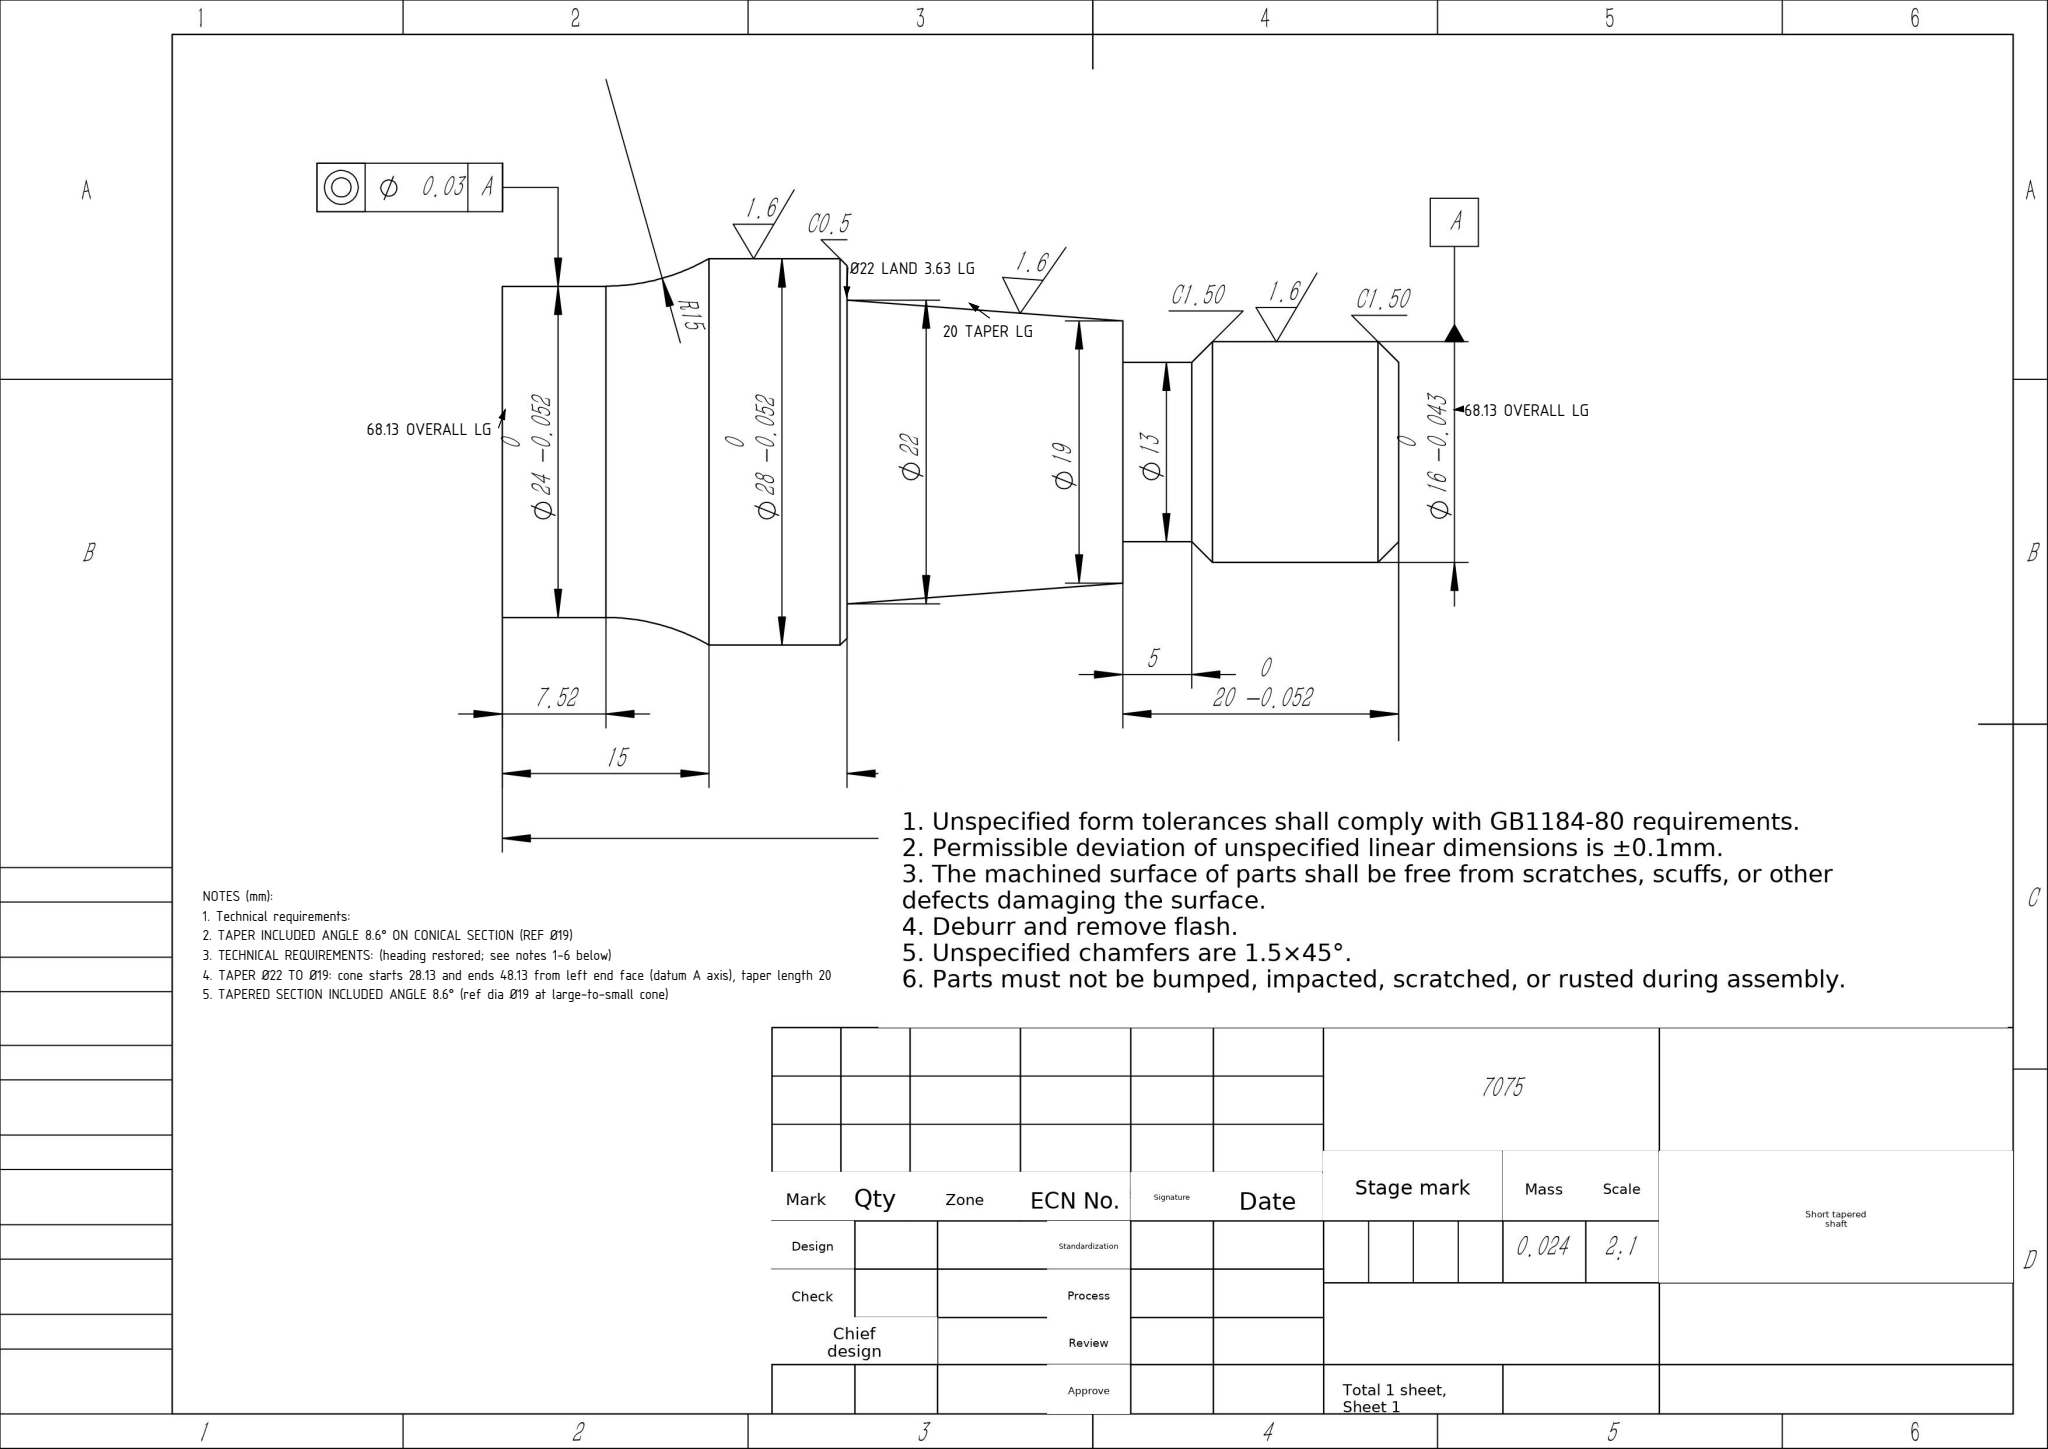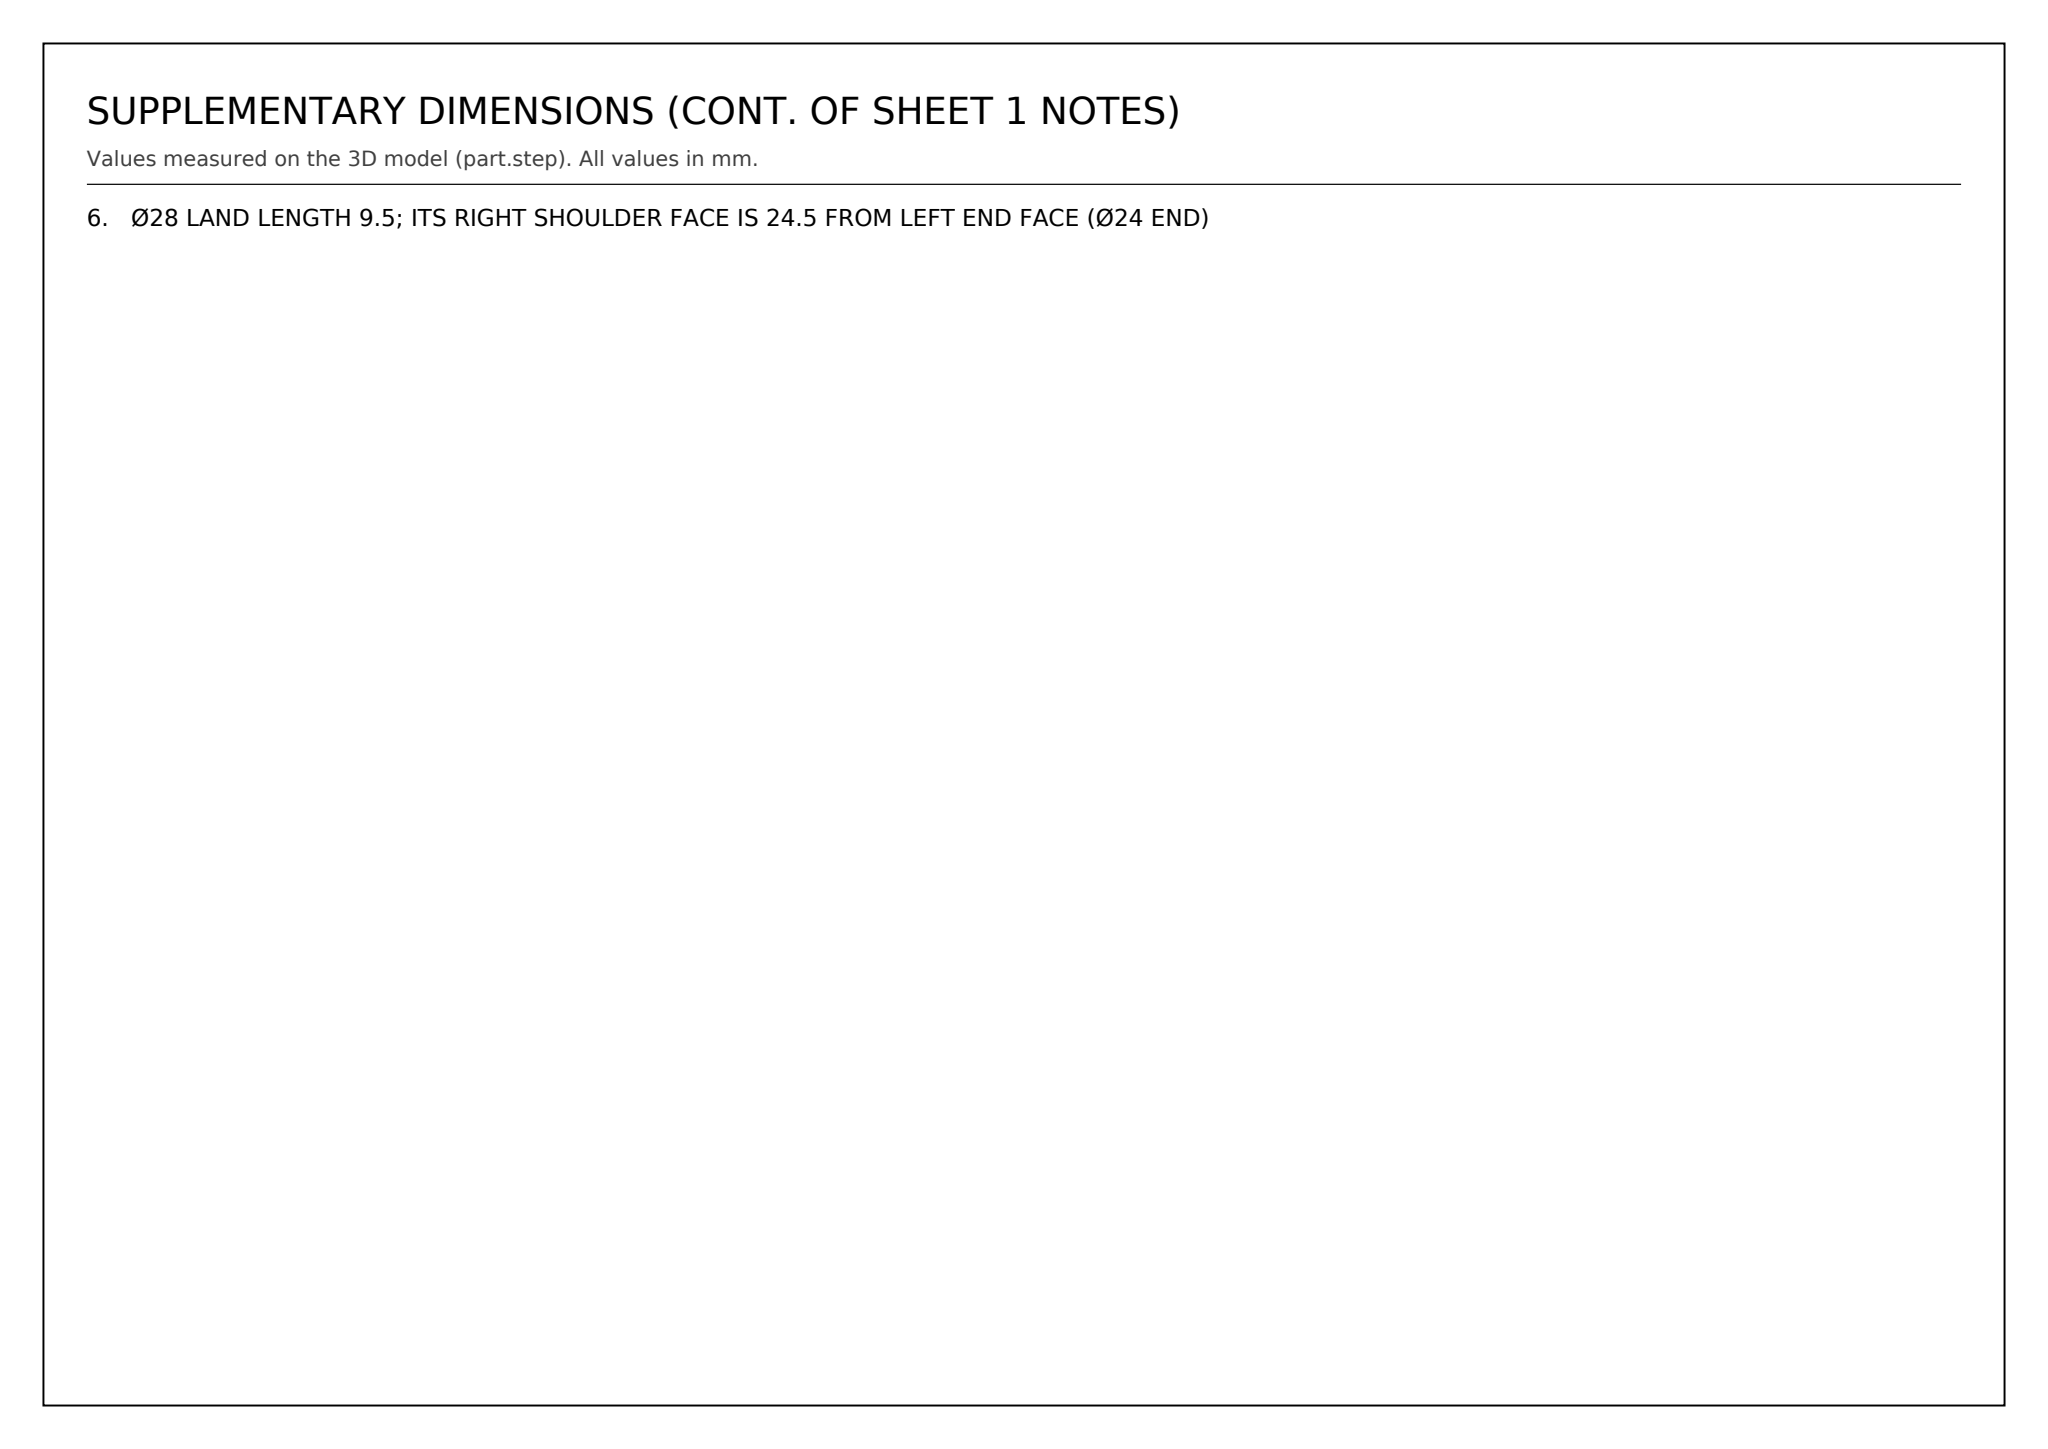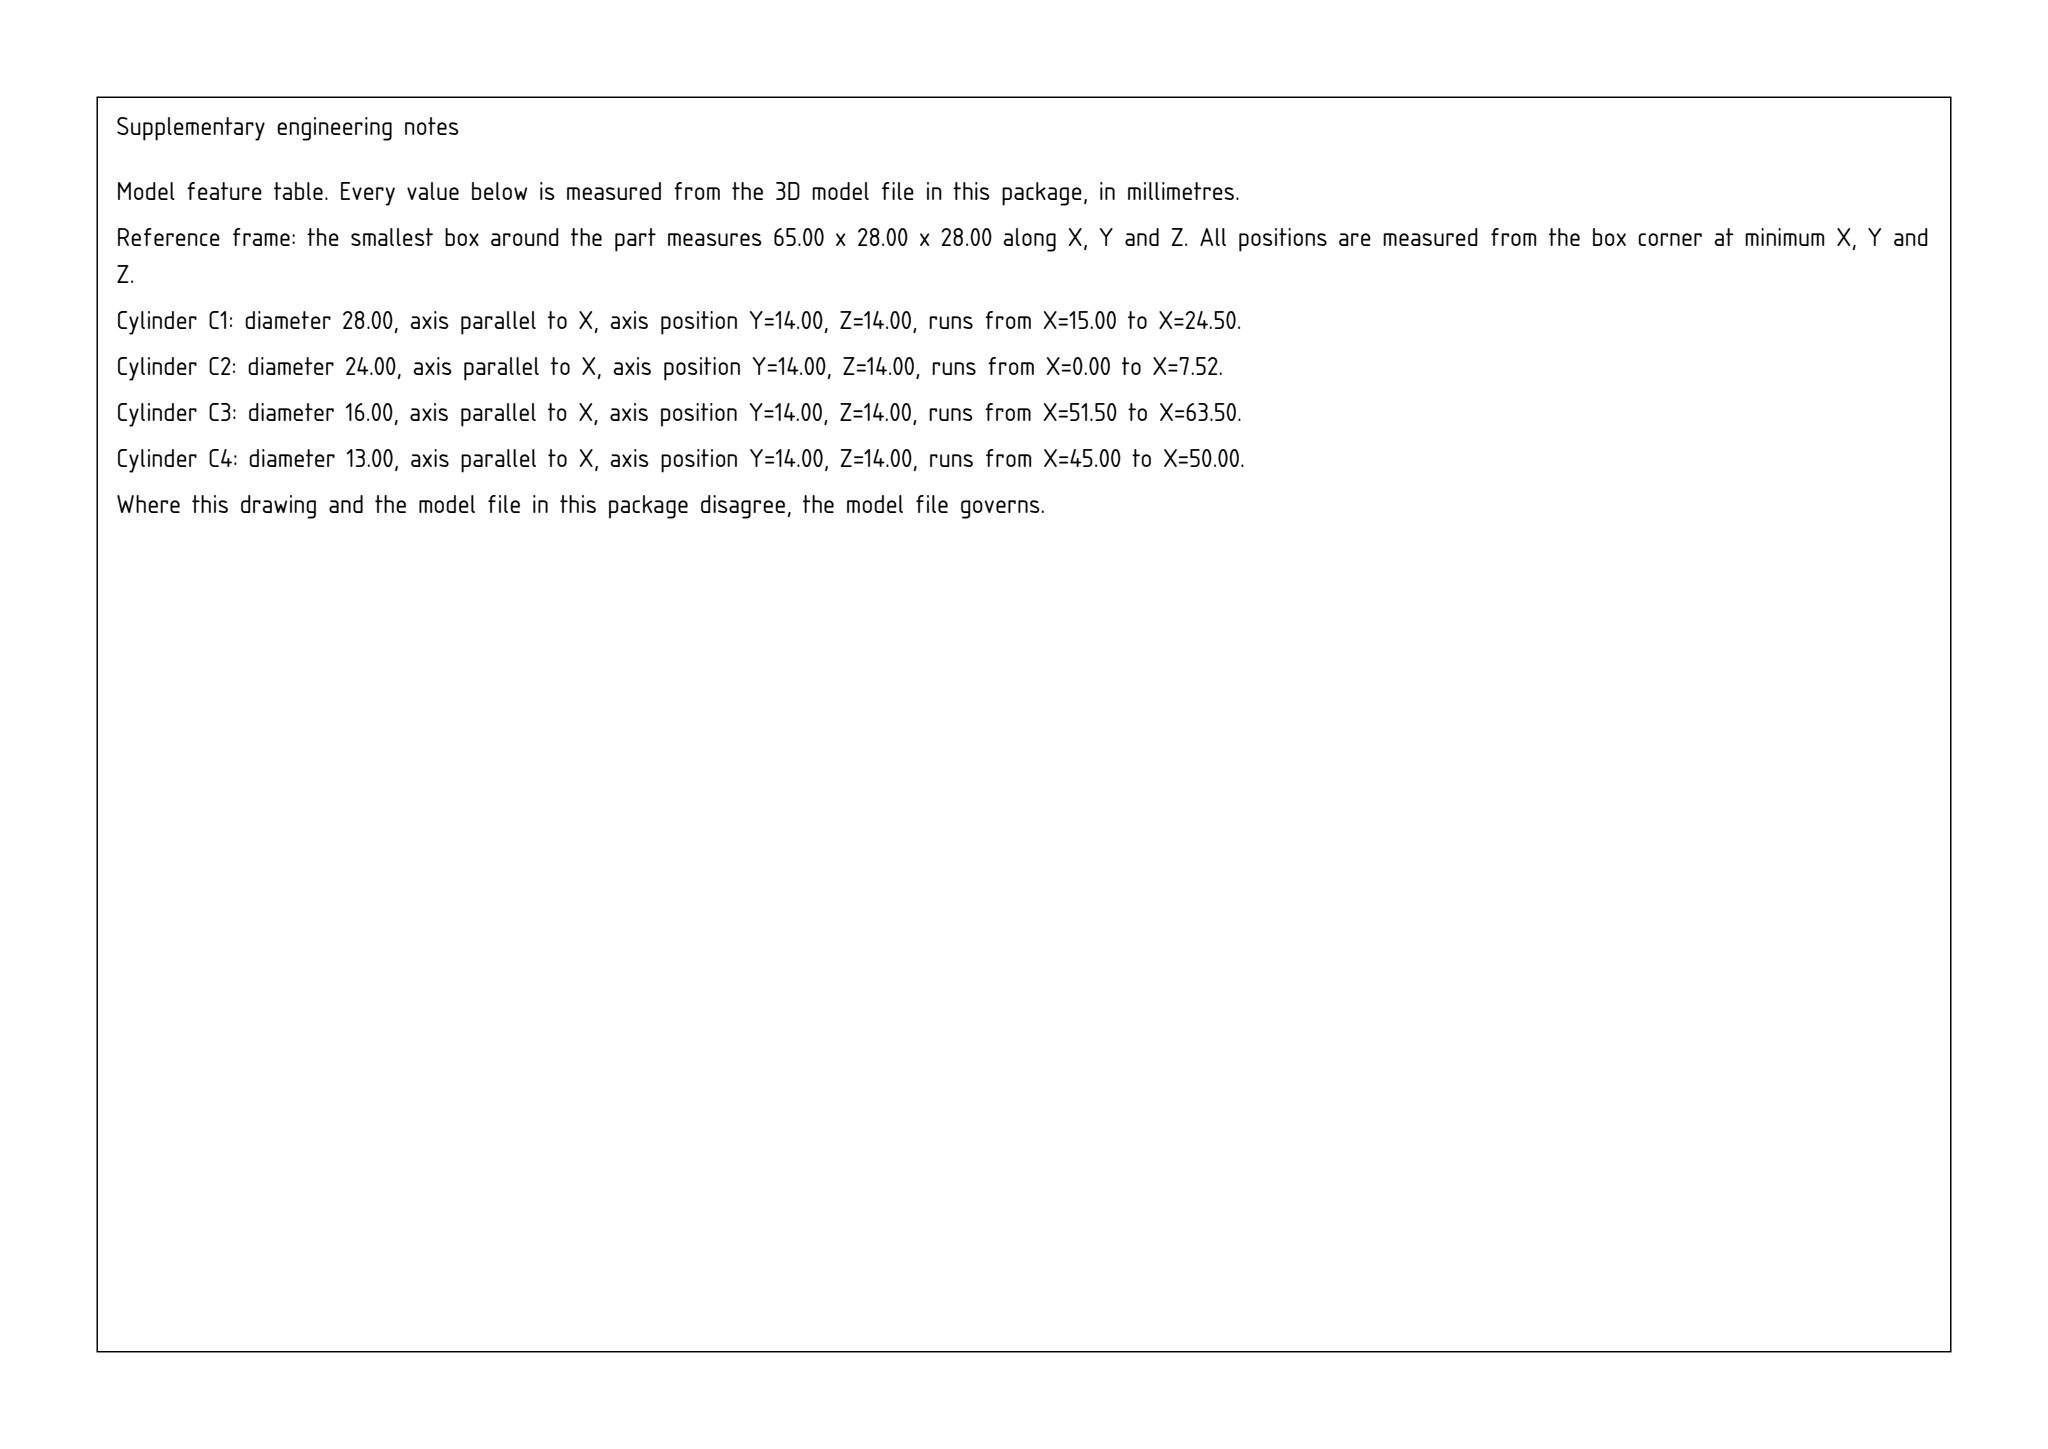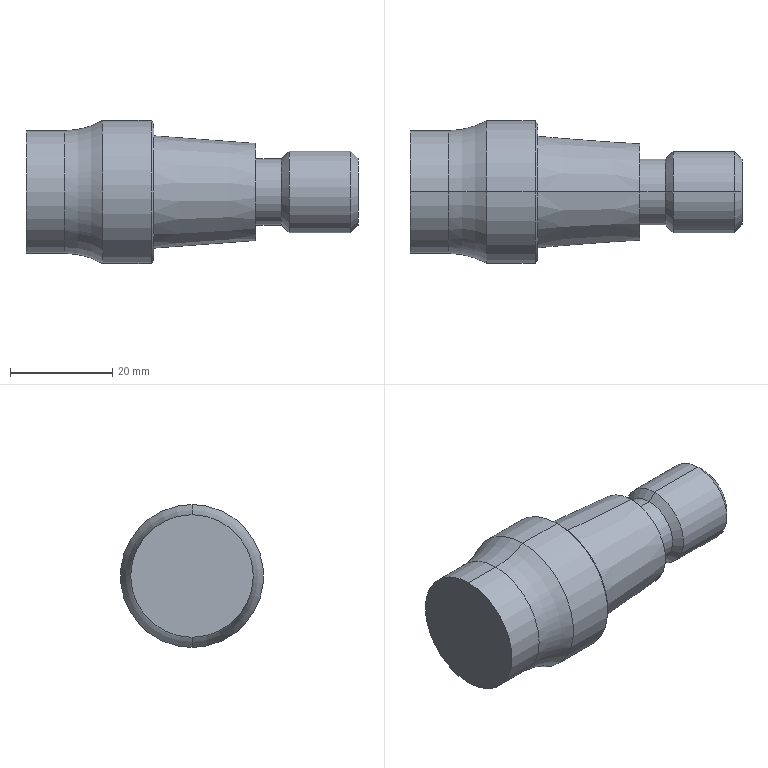Part | SolidWorks | mm | material 7075 | 1 solid | 22 faces | box 65 x 28 x 28 mm | volume 23503 mm3 | cone 8 | cylinder 8 | plane 4 | torus 2 | commonest cylinder face diameters 16 x2 13 x2 28 x2 24 x2
Drawing notes:
Technical requirements: | from the solid: heading text restored after removing merged dimension values (no STEP value)
OVERALL LENGTH 68.13 FROM LEFT END FACE (Ø24 END) TO RIGHT END FACE | from the solid: bbox_xyz x = 68.133; axis_planes x offsets 3.13 ... 68.13
TAPERED SECTION Ø22 TO Ø19: AXIAL LENGTH 20, STARTS 28.13 AND ENDS 48.13 FROM LEFT END FACE | from the solid: axis_planes[x,28.13] and axis_planes[x,48.13]; cone ref_dia 19
TAPER INCLUDED ANGLE 8.6° ON CONICAL SECTION (REF Ø19) | from the solid: cones[included_angle,ref_dia] = [8.6, 19.0]
TECHNICAL REQUIREMENTS: (heading restored; see notes 1-6 below) | from the solid: heading text only - restores garbled line, no dimension value
OVERALL LENGTH 68.13 from left (Ø24) end face to right (Ø16) end face | from the solid: bbox_xyz x = 68.133
TAPER Ø22 TO Ø19: cone starts 28.13 and ends 48.13 from left end face (datum A axis), taper length 20 | from the solid: axis_planes x = 28.13 and x = 48.13 (positions from min corner)
TAPERED SECTION INCLUDED ANGLE 8.6° (ref dia Ø19 at large-to-small cone) | from the solid: cones[included_angle,ref_dia] = [8.6, 19.0]
Ø28 LAND LENGTH 9.5; ITS RIGHT SHOULDER FACE IS 24.5 FROM LEFT END FACE (Ø24 END) | from the solid: cylinders: [28.0,'x',length 9.5] starting 15 from left end face (Ø24 cyl length 7.52 + R15 fillet run), giving shoulder at 24.5
Ø22 LAND FROM 24.5 TO 28.13 FROM LEFT END FACE, LENGTH 3.63, ENDING AT START OF Ø22-TO-Ø19 TAPER | from the solid: axis_planes x=28.13 (cone start) minus Ø28 land end 24.5 (15 + 9.5 Ø28 length)
STEP:
#1=CARTESIAN_POINT('',(25.,0.,-13.5));
#2=VERTEX_POINT('',#1);
#3=CARTESIAN_POINT('',(25.,0.,13.5));
#4=VERTEX_POINT('',#3);
#5=CARTESIAN_POINT('',(25.,0.,0.));
#6=DIRECTION('',(1.,0.,0.));
#7=DIRECTION('',(0.,0.,-1.));
#8=AXIS2_PLACEMENT_3D('',#5,#6,#7);
#9=CIRCLE('',#8,13.5);
#10=EDGE_CURVE('',#2,#4,#9,.T.);
#11=ORIENTED_EDGE('',*,*,#10,.F.);
#12=CARTESIAN_POINT('',(24.5,0.,-14.));
#13=VERTEX_POINT('',#12);
#14=CARTESIAN_POINT('',(25.,0.,-13.5));
#15=DIRECTION('',(-0.7071,0.,-0.7071));
#16=VECTOR('',#15,1000.);
#17=LINE('',#14,#16);
#18=EDGE_CURVE('',#2,#13,#17,.T.);
#19=ORIENTED_EDGE('',*,*,#18,.T.);
#20=CARTESIAN_POINT('',(24.5,0.,14.));
#21=VERTEX_POINT('',#20);
#22=CARTESIAN_POINT('',(24.5,0.,0.));
#23=DIRECTION('',(-1.,0.,0.));
#24=DIRECTION('',(0.,0.,-1.));
#25=AXIS2_PLACEMENT_3D('',#22,#23,#24);
#26=CIRCLE('',#25,14.);
#27=EDGE_CURVE('',#21,#13,#26,.T.);
#28=ORIENTED_EDGE('',*,*,#27,.F.);
#29=CARTESIAN_POINT('',(25.,0.,13.5));
#30=DIRECTION('',(-0.7071,0.,0.7071));
#31=VECTOR('',#30,1000.);
#32=LINE('',#29,#31);
#33=EDGE_CURVE('',#4,#21,#32,.T.);
#34=ORIENTED_EDGE('',*,*,#33,.F.);
#35=EDGE_LOOP('',(#11,#19,#28,#34));
#36=FACE_OUTER_BOUND('',#35,.T.);
#37=CARTESIAN_POINT('',(25.,0.,0.));
#38=DIRECTION('',(-1.,0.,0.));
#39=DIRECTION('',(0.,0.,1.));
#40=AXIS2_PLACEMENT_3D('',#37,#38,#39);
#41=CONICAL_SURFACE('',#40,13.5,0.7854);
#42=ADVANCED_FACE('',(#36),#41,.T.);
#43=CARTESIAN_POINT('',(65.,0.,-6.5));
#44=VERTEX_POINT('',#43);
#45=CARTESIAN_POINT('',(65.,0.,6.5));
#46=VERTEX_POINT('',#45);
#47=CARTESIAN_POINT('',(65.,0.,0.));
#48=DIRECTION('',(1.,0.,0.));
#49=DIRECTION('',(0.,0.,-1.));
#50=AXIS2_PLACEMENT_3D('',#47,#48,#49);
#51=CIRCLE('',#50,6.5);
#52=EDGE_CURVE('',#44,#46,#51,.T.);
#53=ORIENTED_EDGE('',*,*,#52,.F.);
#54=CARTESIAN_POINT('',(63.5,0.,-8.));
#55=VERTEX_POINT('',#54);
#56=CARTESIAN_POINT('',(65.,0.,-6.5));
#57=DIRECTION('',(-0.7071,0.,-0.7071));
#58=VECTOR('',#57,1000.);
#59=LINE('',#56,#58);
#60=EDGE_CURVE('',#44,#55,#59,.T.);
#61=ORIENTED_EDGE('',*,*,#60,.T.);
#62=CARTESIAN_POINT('',(63.5,0.,8.));
#63=VERTEX_POINT('',#62);
#64=CARTESIAN_POINT('',(63.5,0.,0.));
#65=DIRECTION('',(-1.,0.,0.));
#66=DIRECTION('',(0.,0.,-1.));
#67=AXIS2_PLACEMENT_3D('',#64,#65,#66);
#68=CIRCLE('',#67,8.);
#69=EDGE_CURVE('',#63,#55,#68,.T.);
#70=ORIENTED_EDGE('',*,*,#69,.F.);
#71=CARTESIAN_POINT('',(65.,0.,6.5));
#72=DIRECTION('',(-0.7071,0.,0.7071));
#73=VECTOR('',#72,1000.);
#74=LINE('',#71,#73);
#75=EDGE_CURVE('',#46,#63,#74,.T.);
#76=ORIENTED_EDGE('',*,*,#75,.F.);
#77=EDGE_LOOP('',(#53,#61,#70,#76));
#78=FACE_OUTER_BOUND('',#77,.T.);
#79=CARTESIAN_POINT('',(65.,0.,0.));
#80=DIRECTION('',(-1.,0.,0.));
#81=DIRECTION('',(0.,0.,1.));
#82=AXIS2_PLACEMENT_3D('',#79,#80,#81);
#83=CONICAL_SURFACE('',#82,6.5,0.7854);
#84=ADVANCED_FACE('',(#78),#83,.T.);
#85=CARTESIAN_POINT('',(50.,0.,-6.5));
#86=VERTEX_POINT('',#85);
#87=CARTESIAN_POINT('',(50.,0.,6.5));
#88=VERTEX_POINT('',#87);
#89=CARTESIAN_POINT('',(50.,0.,0.));
#90=DIRECTION('',(1.,0.,0.));
#91=DIRECTION('',(0.,0.,-1.));
#92=AXIS2_PLACEMENT_3D('',#89,#90,#91);
#93=CIRCLE('',#92,6.5);
#94=EDGE_CURVE('',#86,#88,#93,.T.);
#95=ORIENTED_EDGE('',*,*,#94,.T.);
#96=CARTESIAN_POINT('',(51.5,0.,8.));
#97=VERTEX_POINT('',#96);
#98=CARTESIAN_POINT('',(51.5,0.,8.));
#99=DIRECTION('',(0.7071,0.,0.7071));
#100=VECTOR('',#99,1000.);
#101=LINE('',#98,#100);
#102=EDGE_CURVE('',#88,#97,#101,.T.);
#103=ORIENTED_EDGE('',*,*,#102,.T.);
#104=CARTESIAN_POINT('',(51.5,0.,-8.));
#105=VERTEX_POINT('',#104);
#106=CARTESIAN_POINT('',(51.5,0.,0.));
#107=DIRECTION('',(1.,0.,0.));
#108=DIRECTION('',(0.,0.,1.));
#109=AXIS2_PLACEMENT_3D('',#106,#107,#108);
#110=CIRCLE('',#109,8.);
#111=EDGE_CURVE('',#105,#97,#110,.T.);
#112=ORIENTED_EDGE('',*,*,#111,.F.);
#113=CARTESIAN_POINT('',(51.5,0.,-8.));
#114=DIRECTION('',(0.7071,0.,-0.7071));
#115=VECTOR('',#114,1000.);
#116=LINE('',#113,#115);
#117=EDGE_CURVE('',#86,#105,#116,.T.);
#118=ORIENTED_EDGE('',*,*,#117,.F.);
#119=EDGE_LOOP('',(#95,#103,#112,#118));
#120=FACE_OUTER_BOUND('',#119,.T.);
#121=CARTESIAN_POINT('',(51.5,0.,0.));
#122=DIRECTION('',(1.,0.,0.));
#123=DIRECTION('',(0.,0.,-1.));
#124=AXIS2_PLACEMENT_3D('',#121,#122,#123);
#125=CONICAL_SURFACE('',#124,8.,0.7854);
#126=ADVANCED_FACE('',(#120),#125,.T.);
#127=ORIENTED_EDGE('',*,*,#111,.T.);
#128=CARTESIAN_POINT('',(65.,0.,8.));
#129=DIRECTION('',(1.,0.,0.));
#130=VECTOR('',#129,1000.);
#131=LINE('',#128,#130);
#132=EDGE_CURVE('',#97,#63,#131,.T.);
#133=ORIENTED_EDGE('',*,*,#132,.T.);
#134=ORIENTED_EDGE('',*,*,#69,.T.);
#135=CARTESIAN_POINT('',(65.,0.,-8.));
#136=DIRECTION('',(1.,0.,0.));
#137=VECTOR('',#136,1000.);
#138=LINE('',#135,#137);
#139=EDGE_CURVE('',#105,#55,#138,.T.);
#140=ORIENTED_EDGE('',*,*,#139,.F.);
#141=EDGE_LOOP('',(#127,#133,#134,#140));
#142=FACE_OUTER_BOUND('',#141,.T.);
#143=CARTESIAN_POINT('',(65.,0.,0.));
#144=DIRECTION('',(1.,0.,0.));
#145=DIRECTION('',(0.,0.,-1.));
#146=AXIS2_PLACEMENT_3D('',#143,#144,#145);
#147=CYLINDRICAL_SURFACE('',#146,8.);
#148=ADVANCED_FACE('',(#142),#147,.T.);
#149=CARTESIAN_POINT('',(45.,0.,-6.5));
#150=VERTEX_POINT('',#149);
#151=CARTESIAN_POINT('',(45.,0.,6.5));
#152=VERTEX_POINT('',#151);
#153=CARTESIAN_POINT('',(45.,0.,0.));
#154=DIRECTION('',(1.,0.,0.));
#155=DIRECTION('',(0.,0.,-1.));
#156=AXIS2_PLACEMENT_3D('',#153,#154,#155);
#157=CIRCLE('',#156,6.5);
#158=EDGE_CURVE('',#150,#152,#157,.T.);
#159=ORIENTED_EDGE('',*,*,#158,.T.);
#160=CARTESIAN_POINT('',(65.,0.,6.5));
#161=DIRECTION('',(1.,0.,0.));
#162=VECTOR('',#161,1000.);
#163=LINE('',#160,#162);
#164=EDGE_CURVE('',#152,#88,#163,.T.);
#165=ORIENTED_EDGE('',*,*,#164,.T.);
#166=ORIENTED_EDGE('',*,*,#94,.F.);
#167=CARTESIAN_POINT('',(65.,0.,-6.5));
#168=DIRECTION('',(1.,0.,0.));
#169=VECTOR('',#168,1000.);
#170=LINE('',#167,#169);
#171=EDGE_CURVE('',#150,#86,#170,.T.);
#172=ORIENTED_EDGE('',*,*,#171,.F.);
#173=EDGE_LOOP('',(#159,#165,#166,#172));
#174=FACE_OUTER_BOUND('',#173,.T.);
#175=CARTESIAN_POINT('',(65.,0.,0.));
#176=DIRECTION('',(1.,0.,0.));
#177=DIRECTION('',(0.,0.,-1.));
#178=AXIS2_PLACEMENT_3D('',#175,#176,#177);
#179=CYLINDRICAL_SURFACE('',#178,6.5);
#180=ADVANCED_FACE('',(#174),#179,.T.);
#181=CARTESIAN_POINT('',(45.,0.,-9.5));
#182=VERTEX_POINT('',#181);
#183=CARTESIAN_POINT('',(45.,0.,9.5));
#184=VERTEX_POINT('',#183);
#185=CARTESIAN_POINT('',(45.,0.,0.));
#186=DIRECTION('',(1.,0.,0.));
#187=DIRECTION('',(0.,0.,-1.));
#188=AXIS2_PLACEMENT_3D('',#185,#186,#187);
#189=CIRCLE('',#188,9.5);
#190=EDGE_CURVE('',#182,#184,#189,.T.);
#191=ORIENTED_EDGE('',*,*,#190,.F.);
#192=CARTESIAN_POINT('',(25.,0.,-11.));
#193=VERTEX_POINT('',#192);
#194=CARTESIAN_POINT('',(45.,0.,-9.5));
#195=DIRECTION('',(-0.9972,0.,-0.07479));
#196=VECTOR('',#195,1000.);
#197=LINE('',#194,#196);
#198=EDGE_CURVE('',#182,#193,#197,.T.);
#199=ORIENTED_EDGE('',*,*,#198,.T.);
#200=CARTESIAN_POINT('',(25.,0.,11.));
#201=VERTEX_POINT('',#200);
#202=CARTESIAN_POINT('',(25.,0.,0.));
#203=DIRECTION('',(1.,0.,0.));
#204=DIRECTION('',(0.,0.,-1.));
#205=AXIS2_PLACEMENT_3D('',#202,#203,#204);
#206=CIRCLE('',#205,11.);
#207=EDGE_CURVE('',#193,#201,#206,.T.);
#208=ORIENTED_EDGE('',*,*,#207,.T.);
#209=CARTESIAN_POINT('',(45.,0.,9.5));
#210=DIRECTION('',(-0.9972,0.,0.07479));
#211=VECTOR('',#210,1000.);
#212=LINE('',#209,#211);
#213=EDGE_CURVE('',#184,#201,#212,.T.);
#214=ORIENTED_EDGE('',*,*,#213,.F.);
#215=EDGE_LOOP('',(#191,#199,#208,#214));
#216=FACE_OUTER_BOUND('',#215,.T.);
#217=CARTESIAN_POINT('',(45.,0.,0.));
#218=DIRECTION('',(-1.,0.,0.));
#219=DIRECTION('',(0.,0.,1.));
#220=AXIS2_PLACEMENT_3D('',#217,#218,#219);
#221=CONICAL_SURFACE('',#220,9.5,0.07486);
#222=ADVANCED_FACE('',(#216),#221,.T.);
#223=CARTESIAN_POINT('',(15.,0.,-14.));
#224=VERTEX_POINT('',#223);
#225=CARTESIAN_POINT('',(15.,0.,14.));
#226=VERTEX_POINT('',#225);
#227=CARTESIAN_POINT('',(15.,0.,0.));
#228=DIRECTION('',(1.,0.,0.));
#229=DIRECTION('',(0.,0.,-1.));
#230=AXIS2_PLACEMENT_3D('',#227,#228,#229);
#231=CIRCLE('',#230,14.);
#232=EDGE_CURVE('',#224,#226,#231,.T.);
#233=ORIENTED_EDGE('',*,*,#232,.T.);
#234=CARTESIAN_POINT('',(65.,0.,14.));
#235=DIRECTION('',(1.,0.,0.));
#236=VECTOR('',#235,1000.);
#237=LINE('',#234,#236);
#238=EDGE_CURVE('',#226,#21,#237,.T.);
#239=ORIENTED_EDGE('',*,*,#238,.T.);
#240=ORIENTED_EDGE('',*,*,#27,.T.);
#241=CARTESIAN_POINT('',(65.,0.,-14.));
#242=DIRECTION('',(1.,0.,0.));
#243=VECTOR('',#242,1000.);
#244=LINE('',#241,#243);
#245=EDGE_CURVE('',#224,#13,#244,.T.);
#246=ORIENTED_EDGE('',*,*,#245,.F.);
#247=EDGE_LOOP('',(#233,#239,#240,#246));
#248=FACE_OUTER_BOUND('',#247,.T.);
#249=CARTESIAN_POINT('',(65.,0.,0.));
#250=DIRECTION('',(1.,0.,0.));
#251=DIRECTION('',(0.,0.,-1.));
#252=AXIS2_PLACEMENT_3D('',#249,#250,#251);
#253=CYLINDRICAL_SURFACE('',#252,14.);
#254=ADVANCED_FACE('',(#248),#253,.T.);
#255=CARTESIAN_POINT('',(15.,0.,0.));
#256=DIRECTION('',(1.,0.,0.));
#257=DIRECTION('',(0.,0.,-1.));
#258=AXIS2_PLACEMENT_3D('',#255,#256,#257);
#259=CIRCLE('',#258,14.);
#260=EDGE_CURVE('',#226,#224,#259,.T.);
#261=ORIENTED_EDGE('',*,*,#260,.F.);
#262=CARTESIAN_POINT('',(7.517,0.,12.));
#263=VERTEX_POINT('',#262);
#264=CARTESIAN_POINT('',(7.517,0.,27.));
#265=DIRECTION('',(0.,1.,-0.));
#266=DIRECTION('',(0.,0.,1.));
#267=AXIS2_PLACEMENT_3D('',#264,#265,#266);
#268=CIRCLE('',#267,15.);
#269=EDGE_CURVE('',#226,#263,#268,.T.);
#270=ORIENTED_EDGE('',*,*,#269,.T.);
#271=CARTESIAN_POINT('',(7.517,0.,-12.));
#272=VERTEX_POINT('',#271);
#273=CARTESIAN_POINT('',(7.517,0.,0.));
#274=DIRECTION('',(1.,0.,0.));
#275=DIRECTION('',(0.,0.,-1.));
#276=AXIS2_PLACEMENT_3D('',#273,#274,#275);
#277=CIRCLE('',#276,12.);
#278=EDGE_CURVE('',#263,#272,#277,.T.);
#279=ORIENTED_EDGE('',*,*,#278,.T.);
#280=CARTESIAN_POINT('',(7.517,0.,-27.));
#281=DIRECTION('',(0.,-1.,0.));
#282=DIRECTION('',(0.,0.,-1.));
#283=AXIS2_PLACEMENT_3D('',#280,#281,#282);
#284=CIRCLE('',#283,15.);
#285=EDGE_CURVE('',#224,#272,#284,.T.);
#286=ORIENTED_EDGE('',*,*,#285,.F.);
#287=EDGE_LOOP('',(#261,#270,#279,#286));
#288=FACE_OUTER_BOUND('',#287,.T.);
#289=CARTESIAN_POINT('',(7.517,0.,0.));
#290=DIRECTION('',(1.,0.,0.));
#291=DIRECTION('',(0.,0.,-1.));
#292=AXIS2_PLACEMENT_3D('',#289,#290,#291);
#293=TOROIDAL_SURFACE('',#292,27.,15.);
#294=ADVANCED_FACE('',(#288),#293,.F.);
#295=CARTESIAN_POINT('',(0.,0.,-12.));
#296=VERTEX_POINT('',#295);
#297=CARTESIAN_POINT('',(0.,0.,12.));
#298=VERTEX_POINT('',#297);
#299=CARTESIAN_POINT('',(0.,0.,0.));
#300=DIRECTION('',(1.,0.,0.));
#301=DIRECTION('',(0.,0.,-1.));
#302=AXIS2_PLACEMENT_3D('',#299,#300,#301);
#303=CIRCLE('',#302,12.);
#304=EDGE_CURVE('',#296,#298,#303,.T.);
#305=ORIENTED_EDGE('',*,*,#304,.T.);
#306=CARTESIAN_POINT('',(65.,0.,12.));
#307=DIRECTION('',(1.,0.,0.));
#308=VECTOR('',#307,1000.);
#309=LINE('',#306,#308);
#310=EDGE_CURVE('',#298,#263,#309,.T.);
#311=ORIENTED_EDGE('',*,*,#310,.T.);
#312=CARTESIAN_POINT('',(7.517,0.,0.));
#313=DIRECTION('',(1.,0.,0.));
#314=DIRECTION('',(0.,0.,-1.));
#315=AXIS2_PLACEMENT_3D('',#312,#313,#314);
#316=CIRCLE('',#315,12.);
#317=EDGE_CURVE('',#272,#263,#316,.T.);
#318=ORIENTED_EDGE('',*,*,#317,.F.);
#319=CARTESIAN_POINT('',(65.,0.,-12.));
#320=DIRECTION('',(1.,0.,0.));
#321=VECTOR('',#320,1000.);
#322=LINE('',#319,#321);
#323=EDGE_CURVE('',#296,#272,#322,.T.);
#324=ORIENTED_EDGE('',*,*,#323,.F.);
#325=EDGE_LOOP('',(#305,#311,#318,#324));
#326=FACE_OUTER_BOUND('',#325,.T.);
#327=CARTESIAN_POINT('',(65.,0.,0.));
#328=DIRECTION('',(1.,0.,0.));
#329=DIRECTION('',(0.,0.,-1.));
#330=AXIS2_PLACEMENT_3D('',#327,#328,#329);
#331=CYLINDRICAL_SURFACE('',#330,12.);
#332=ADVANCED_FACE('',(#326),#331,.T.);
#333=ORIENTED_EDGE('',*,*,#304,.F.);
#334=CARTESIAN_POINT('',(0.,0.,0.));
#335=DIRECTION('',(1.,0.,0.));
#336=DIRECTION('',(0.,0.,-1.));
#337=AXIS2_PLACEMENT_3D('',#334,#335,#336);
#338=CIRCLE('',#337,12.);
#339=EDGE_CURVE('',#298,#296,#338,.T.);
#340=ORIENTED_EDGE('',*,*,#339,.F.);
#341=EDGE_LOOP('',(#333,#340));
#342=FACE_OUTER_BOUND('',#341,.T.);
#343=CARTESIAN_POINT('',(0.,0.,0.));
#344=DIRECTION('',(-1.,0.,0.));
#345=DIRECTION('',(0.,0.,1.));
#346=AXIS2_PLACEMENT_3D('',#343,#344,#345);
#347=PLANE('',#346);
#348=ADVANCED_FACE('',(#342),#347,.T.);
#349=ORIENTED_EDGE('',*,*,#310,.F.);
#350=ORIENTED_EDGE('',*,*,#339,.T.);
#351=ORIENTED_EDGE('',*,*,#323,.T.);
#352=ORIENTED_EDGE('',*,*,#278,.F.);
#353=EDGE_LOOP('',(#349,#350,#351,#352));
#354=FACE_OUTER_BOUND('',#353,.T.);
#355=CARTESIAN_POINT('',(65.,0.,0.));
#356=DIRECTION('',(1.,0.,0.));
#357=DIRECTION('',(0.,0.,-1.));
#358=AXIS2_PLACEMENT_3D('',#355,#356,#357);
#359=CYLINDRICAL_SURFACE('',#358,12.);
#360=ADVANCED_FACE('',(#354),#359,.T.);
#361=ORIENTED_EDGE('',*,*,#269,.F.);
#362=ORIENTED_EDGE('',*,*,#232,.F.);
#363=ORIENTED_EDGE('',*,*,#285,.T.);
#364=ORIENTED_EDGE('',*,*,#317,.T.);
#365=EDGE_LOOP('',(#361,#362,#363,#364));
#366=FACE_OUTER_BOUND('',#365,.T.);
#367=CARTESIAN_POINT('',(7.517,0.,0.));
#368=DIRECTION('',(1.,0.,0.));
#369=DIRECTION('',(0.,0.,-1.));
#370=AXIS2_PLACEMENT_3D('',#367,#368,#369);
#371=TOROIDAL_SURFACE('',#370,27.,15.);
#372=ADVANCED_FACE('',(#366),#371,.F.);
#373=ORIENTED_EDGE('',*,*,#238,.F.);
#374=ORIENTED_EDGE('',*,*,#260,.T.);
#375=ORIENTED_EDGE('',*,*,#245,.T.);
#376=CARTESIAN_POINT('',(24.5,0.,0.));
#377=DIRECTION('',(-1.,0.,0.));
#378=DIRECTION('',(0.,0.,-1.));
#379=AXIS2_PLACEMENT_3D('',#376,#377,#378);
#380=CIRCLE('',#379,14.);
#381=EDGE_CURVE('',#13,#21,#380,.T.);
#382=ORIENTED_EDGE('',*,*,#381,.T.);
#383=EDGE_LOOP('',(#373,#374,#375,#382));
#384=FACE_OUTER_BOUND('',#383,.T.);
#385=CARTESIAN_POINT('',(65.,0.,0.));
#386=DIRECTION('',(1.,0.,0.));
#387=DIRECTION('',(0.,0.,-1.));
#388=AXIS2_PLACEMENT_3D('',#385,#386,#387);
#389=CYLINDRICAL_SURFACE('',#388,14.);
#390=ADVANCED_FACE('',(#384),#389,.T.);
#391=CARTESIAN_POINT('',(25.,0.,0.));
#392=DIRECTION('',(1.,0.,0.));
#393=DIRECTION('',(0.,0.,-1.));
#394=AXIS2_PLACEMENT_3D('',#391,#392,#393);
#395=CIRCLE('',#394,13.5);
#396=EDGE_CURVE('',#4,#2,#395,.T.);
#397=ORIENTED_EDGE('',*,*,#396,.T.);
#398=ORIENTED_EDGE('',*,*,#10,.T.);
#399=EDGE_LOOP('',(#397,#398));
#400=FACE_OUTER_BOUND('',#399,.T.);
#401=CARTESIAN_POINT('',(25.,0.,0.));
#402=DIRECTION('',(1.,0.,0.));
#403=DIRECTION('',(0.,0.,-1.));
#404=AXIS2_PLACEMENT_3D('',#401,#402,#403);
#405=CIRCLE('',#404,11.);
#406=EDGE_CURVE('',#201,#193,#405,.T.);
#407=ORIENTED_EDGE('',*,*,#406,.F.);
#408=ORIENTED_EDGE('',*,*,#207,.F.);
#409=EDGE_LOOP('',(#407,#408));
#410=FACE_BOUND('',#409,.T.);
#411=CARTESIAN_POINT('',(25.,14.,0.));
#412=DIRECTION('',(1.,0.,0.));
#413=DIRECTION('',(0.,0.,-1.));
#414=AXIS2_PLACEMENT_3D('',#411,#412,#413);
#415=PLANE('',#414);
#416=ADVANCED_FACE('',(#400,#410),#415,.T.);
#417=ORIENTED_EDGE('',*,*,#198,.F.);
#418=CARTESIAN_POINT('',(45.,0.,0.));
#419=DIRECTION('',(1.,0.,0.));
#420=DIRECTION('',(0.,0.,-1.));
#421=AXIS2_PLACEMENT_3D('',#418,#419,#420);
#422=CIRCLE('',#421,9.5);
#423=EDGE_CURVE('',#184,#182,#422,.T.);
#424=ORIENTED_EDGE('',*,*,#423,.F.);
#425=ORIENTED_EDGE('',*,*,#213,.T.);
#426=ORIENTED_EDGE('',*,*,#406,.T.);
#427=EDGE_LOOP('',(#417,#424,#425,#426));
#428=FACE_OUTER_BOUND('',#427,.T.);
#429=CARTESIAN_POINT('',(45.,0.,0.));
#430=DIRECTION('',(-1.,0.,0.));
#431=DIRECTION('',(0.,0.,1.));
#432=AXIS2_PLACEMENT_3D('',#429,#430,#431);
#433=CONICAL_SURFACE('',#432,9.5,0.07486);
#434=ADVANCED_FACE('',(#428),#433,.T.);
#435=ORIENTED_EDGE('',*,*,#423,.T.);
#436=ORIENTED_EDGE('',*,*,#190,.T.);
#437=EDGE_LOOP('',(#435,#436));
#438=FACE_OUTER_BOUND('',#437,.T.);
#439=ORIENTED_EDGE('',*,*,#158,.F.);
#440=CARTESIAN_POINT('',(45.,0.,0.));
#441=DIRECTION('',(1.,0.,0.));
#442=DIRECTION('',(0.,0.,-1.));
#443=AXIS2_PLACEMENT_3D('',#440,#441,#442);
#444=CIRCLE('',#443,6.5);
#445=EDGE_CURVE('',#152,#150,#444,.T.);
#446=ORIENTED_EDGE('',*,*,#445,.F.);
#447=EDGE_LOOP('',(#439,#446));
#448=FACE_BOUND('',#447,.T.);
#449=CARTESIAN_POINT('',(45.,9.5,0.));
#450=DIRECTION('',(1.,0.,0.));
#451=DIRECTION('',(0.,0.,-1.));
#452=AXIS2_PLACEMENT_3D('',#449,#450,#451);
#453=PLANE('',#452);
#454=ADVANCED_FACE('',(#438,#448),#453,.T.);
#455=ORIENTED_EDGE('',*,*,#164,.F.);
#456=ORIENTED_EDGE('',*,*,#445,.T.);
#457=ORIENTED_EDGE('',*,*,#171,.T.);
#458=CARTESIAN_POINT('',(50.,0.,0.));
#459=DIRECTION('',(1.,0.,0.));
#460=DIRECTION('',(0.,0.,-1.));
#461=AXIS2_PLACEMENT_3D('',#458,#459,#460);
#462=CIRCLE('',#461,6.5);
#463=EDGE_CURVE('',#88,#86,#462,.T.);
#464=ORIENTED_EDGE('',*,*,#463,.F.);
#465=EDGE_LOOP('',(#455,#456,#457,#464));
#466=FACE_OUTER_BOUND('',#465,.T.);
#467=CARTESIAN_POINT('',(65.,0.,0.));
#468=DIRECTION('',(1.,0.,0.));
#469=DIRECTION('',(0.,0.,-1.));
#470=AXIS2_PLACEMENT_3D('',#467,#468,#469);
#471=CYLINDRICAL_SURFACE('',#470,6.5);
#472=ADVANCED_FACE('',(#466),#471,.T.);
#473=ORIENTED_EDGE('',*,*,#132,.F.);
#474=CARTESIAN_POINT('',(51.5,0.,0.));
#475=DIRECTION('',(1.,0.,0.));
#476=DIRECTION('',(0.,0.,1.));
#477=AXIS2_PLACEMENT_3D('',#474,#475,#476);
#478=CIRCLE('',#477,8.);
#479=EDGE_CURVE('',#97,#105,#478,.T.);
#480=ORIENTED_EDGE('',*,*,#479,.T.);
#481=ORIENTED_EDGE('',*,*,#139,.T.);
#482=CARTESIAN_POINT('',(63.5,0.,0.));
#483=DIRECTION('',(-1.,0.,0.));
#484=DIRECTION('',(0.,0.,-1.));
#485=AXIS2_PLACEMENT_3D('',#482,#483,#484);
#486=CIRCLE('',#485,8.);
#487=EDGE_CURVE('',#55,#63,#486,.T.);
#488=ORIENTED_EDGE('',*,*,#487,.T.);
#489=EDGE_LOOP('',(#473,#480,#481,#488));
#490=FACE_OUTER_BOUND('',#489,.T.);
#491=CARTESIAN_POINT('',(65.,0.,0.));
#492=DIRECTION('',(1.,0.,0.));
#493=DIRECTION('',(0.,0.,-1.));
#494=AXIS2_PLACEMENT_3D('',#491,#492,#493);
#495=CYLINDRICAL_SURFACE('',#494,8.);
#496=ADVANCED_FACE('',(#490),#495,.T.);
#497=CARTESIAN_POINT('',(65.,0.,0.));
#498=DIRECTION('',(1.,0.,0.));
#499=DIRECTION('',(0.,0.,-1.));
#500=AXIS2_PLACEMENT_3D('',#497,#498,#499);
#501=CIRCLE('',#500,6.5);
#502=EDGE_CURVE('',#46,#44,#501,.T.);
#503=ORIENTED_EDGE('',*,*,#502,.T.);
#504=ORIENTED_EDGE('',*,*,#52,.T.);
#505=EDGE_LOOP('',(#503,#504));
#506=FACE_OUTER_BOUND('',#505,.T.);
#507=CARTESIAN_POINT('',(65.,8.,0.));
#508=DIRECTION('',(1.,0.,0.));
#509=DIRECTION('',(0.,0.,-1.));
#510=AXIS2_PLACEMENT_3D('',#507,#508,#509);
#511=PLANE('',#510);
#512=ADVANCED_FACE('',(#506),#511,.T.);
#513=ORIENTED_EDGE('',*,*,#102,.F.);
#514=ORIENTED_EDGE('',*,*,#463,.T.);
#515=ORIENTED_EDGE('',*,*,#117,.T.);
#516=ORIENTED_EDGE('',*,*,#479,.F.);
#517=EDGE_LOOP('',(#513,#514,#515,#516));
#518=FACE_OUTER_BOUND('',#517,.T.);
#519=CARTESIAN_POINT('',(51.5,0.,0.));
#520=DIRECTION('',(1.,0.,0.));
#521=DIRECTION('',(0.,0.,-1.));
#522=AXIS2_PLACEMENT_3D('',#519,#520,#521);
#523=CONICAL_SURFACE('',#522,8.,0.7854);
#524=ADVANCED_FACE('',(#518),#523,.T.);
#525=ORIENTED_EDGE('',*,*,#60,.F.);
#526=ORIENTED_EDGE('',*,*,#502,.F.);
#527=ORIENTED_EDGE('',*,*,#75,.T.);
#528=ORIENTED_EDGE('',*,*,#487,.F.);
#529=EDGE_LOOP('',(#525,#526,#527,#528));
#530=FACE_OUTER_BOUND('',#529,.T.);
#531=CARTESIAN_POINT('',(65.,0.,0.));
#532=DIRECTION('',(-1.,0.,0.));
#533=DIRECTION('',(0.,0.,1.));
#534=AXIS2_PLACEMENT_3D('',#531,#532,#533);
#535=CONICAL_SURFACE('',#534,6.5,0.7854);
#536=ADVANCED_FACE('',(#530),#535,.T.);
#537=ORIENTED_EDGE('',*,*,#18,.F.);
#538=ORIENTED_EDGE('',*,*,#396,.F.);
#539=ORIENTED_EDGE('',*,*,#33,.T.);
#540=ORIENTED_EDGE('',*,*,#381,.F.);
#541=EDGE_LOOP('',(#537,#538,#539,#540));
#542=FACE_OUTER_BOUND('',#541,.T.);
#543=CARTESIAN_POINT('',(25.,0.,0.));
#544=DIRECTION('',(-1.,0.,0.));
#545=DIRECTION('',(0.,0.,1.));
#546=AXIS2_PLACEMENT_3D('',#543,#544,#545);
#547=CONICAL_SURFACE('',#546,13.5,0.7854);
#548=ADVANCED_FACE('',(#542),#547,.T.);
#549=CLOSED_SHELL('',(#42,#84,#126,#148,#180,#222,#254,#294,#332,#348,#360,#372,#390,#416,#434,#454,#472,#496,#512,#524,#536,#548));
#550=MANIFOLD_SOLID_BREP('',#549);
#551=CARTESIAN_POINT('',(0.,0.,0.));
#552=DIRECTION('',(0.,0.,1.));
#553=DIRECTION('',(1.,0.,0.));
#554=AXIS2_PLACEMENT_3D('',#551,#552,#553);
#555=(LENGTH_UNIT()NAMED_UNIT(*)SI_UNIT(.MILLI.,.METRE.));
#556=UNCERTAINTY_MEASURE_WITH_UNIT(LENGTH_MEASURE(0.00001),#555,'','');
#557=(NAMED_UNIT(*)PLANE_ANGLE_UNIT()SI_UNIT($,.RADIAN.));
#558=(NAMED_UNIT(*)SI_UNIT($,.STERADIAN.)SOLID_ANGLE_UNIT());
#559=(GEOMETRIC_REPRESENTATION_CONTEXT(3)GLOBAL_UNCERTAINTY_ASSIGNED_CONTEXT((#556))GLOBAL_UNIT_ASSIGNED_CONTEXT((#555,#557,#558))REPRESENTATION_CONTEXT('',''));
#560=ADVANCED_BREP_SHAPE_REPRESENTATION('',(#550,#554),#559);